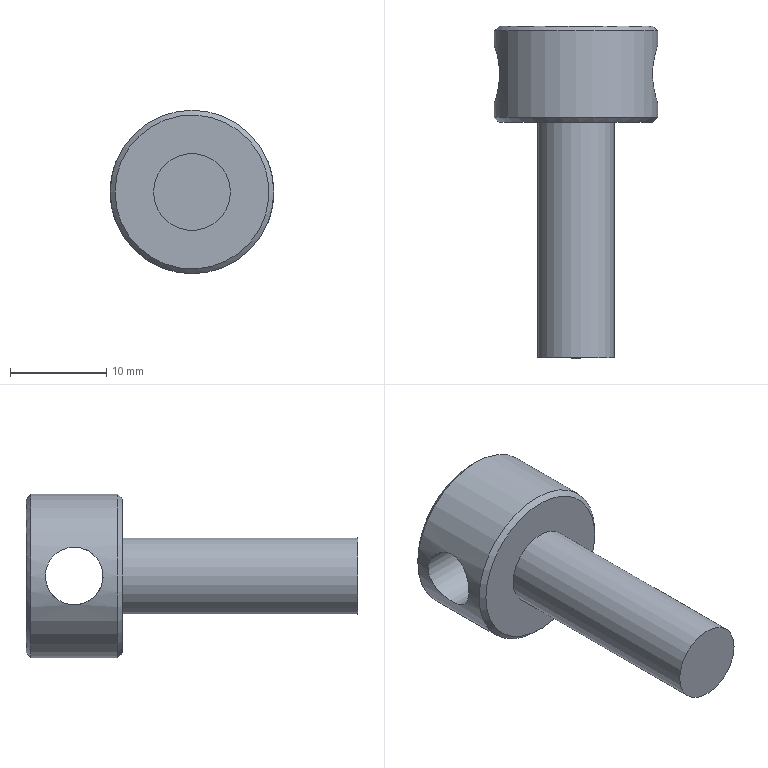Component | NX | THREADED_ROD | 1 solid | 8 faces | volume 3015 mm3 | cylinder 3 | plane 3 | cone 2 | commonest cylinder face diameters 17 x1 8 x1 6 x1